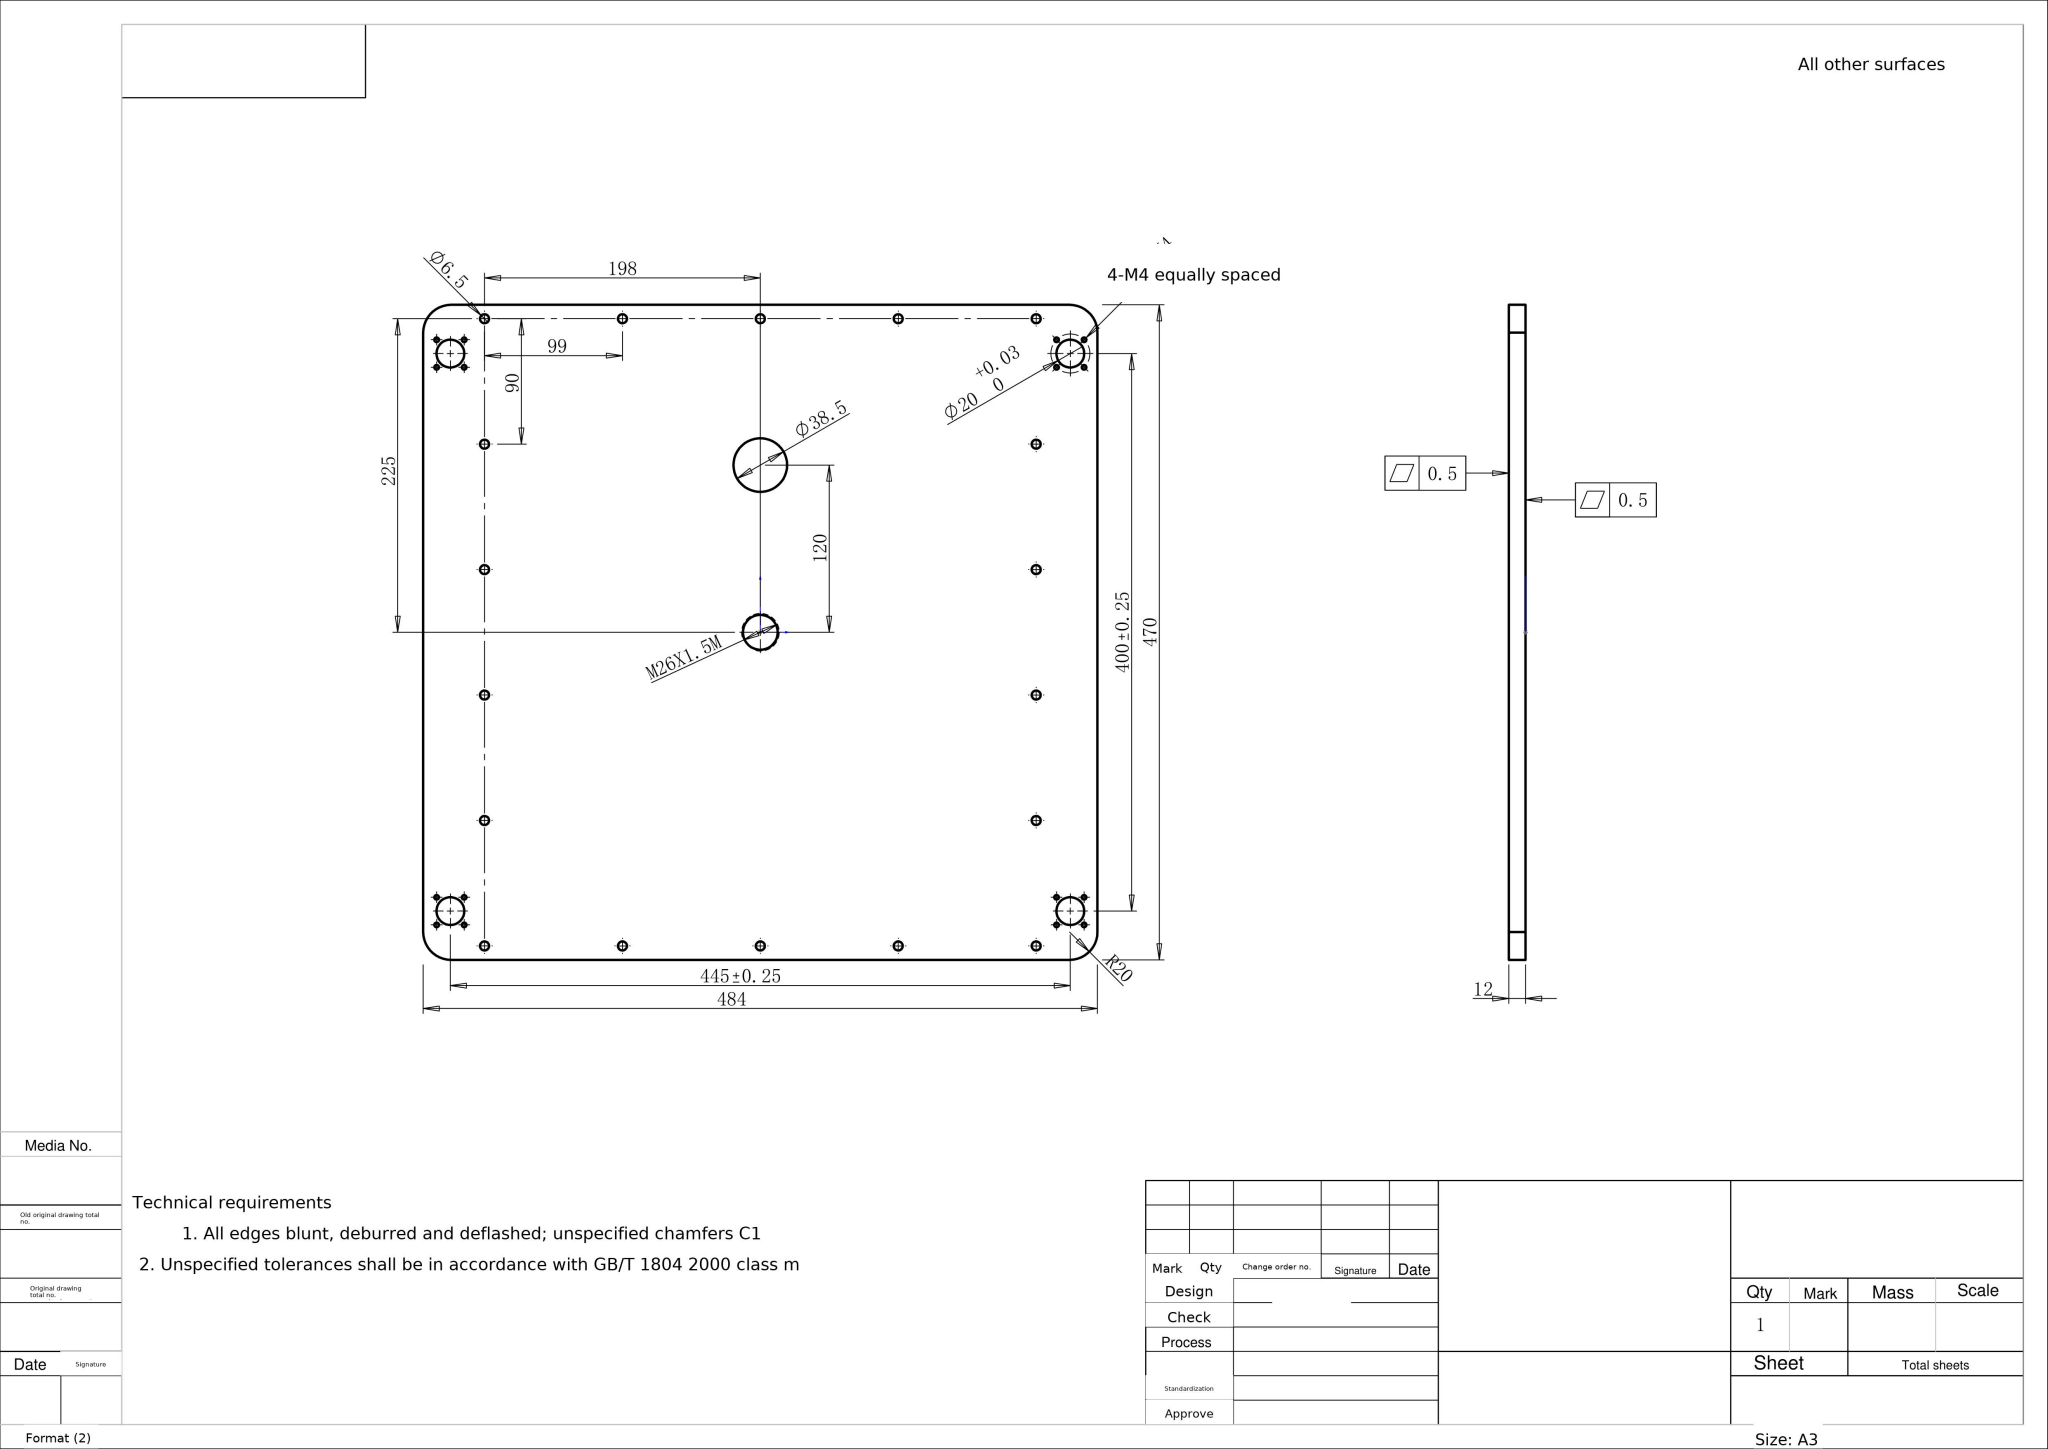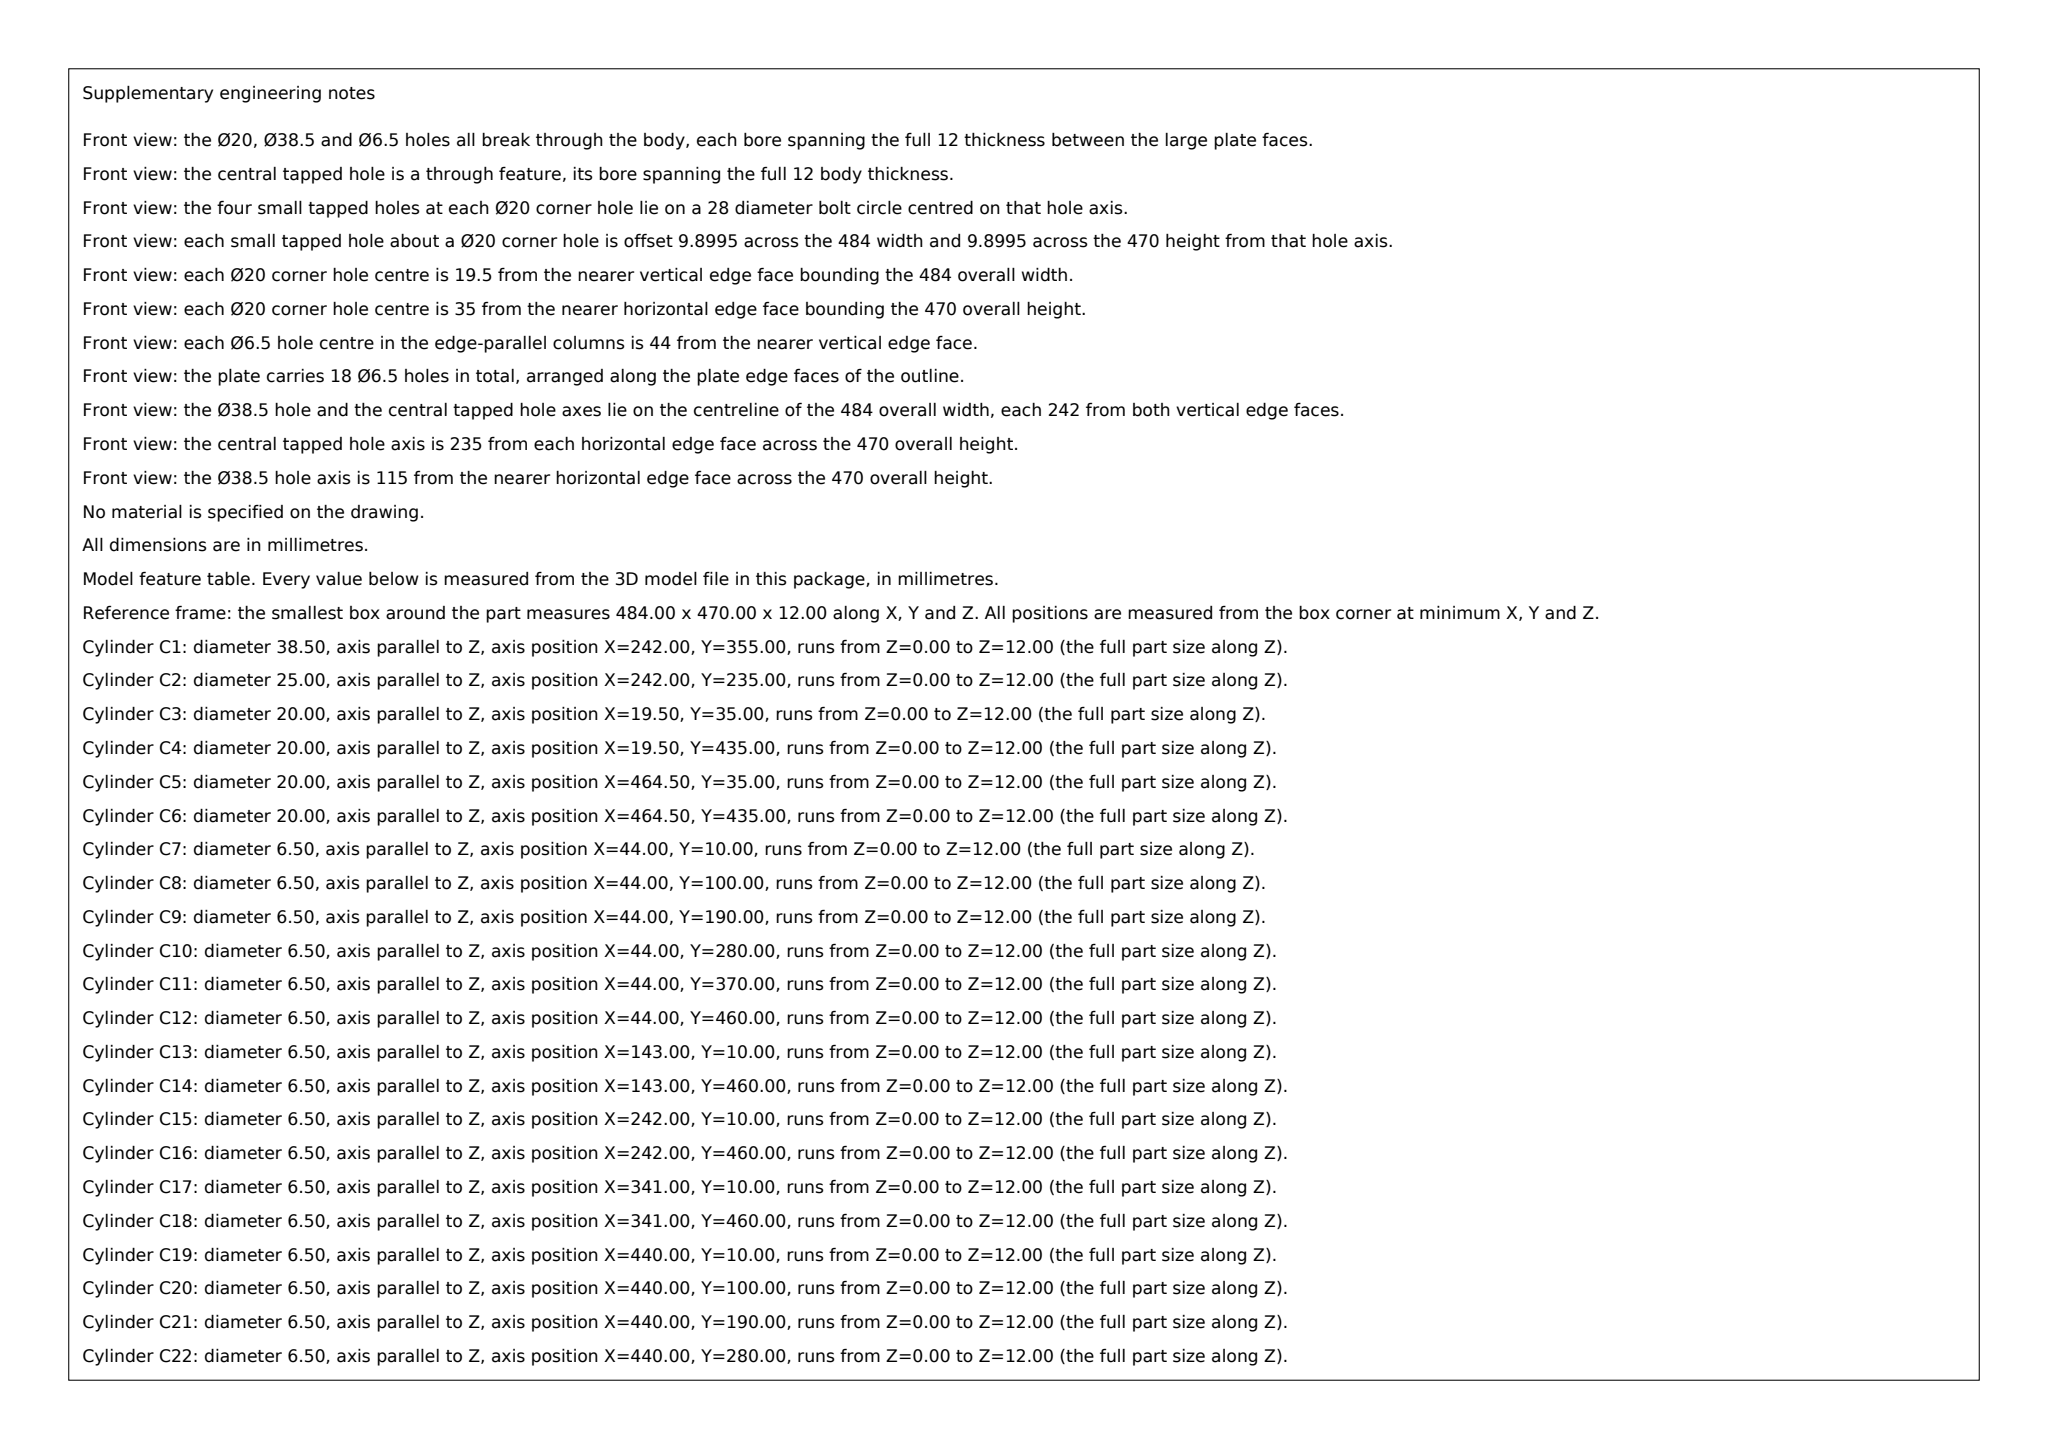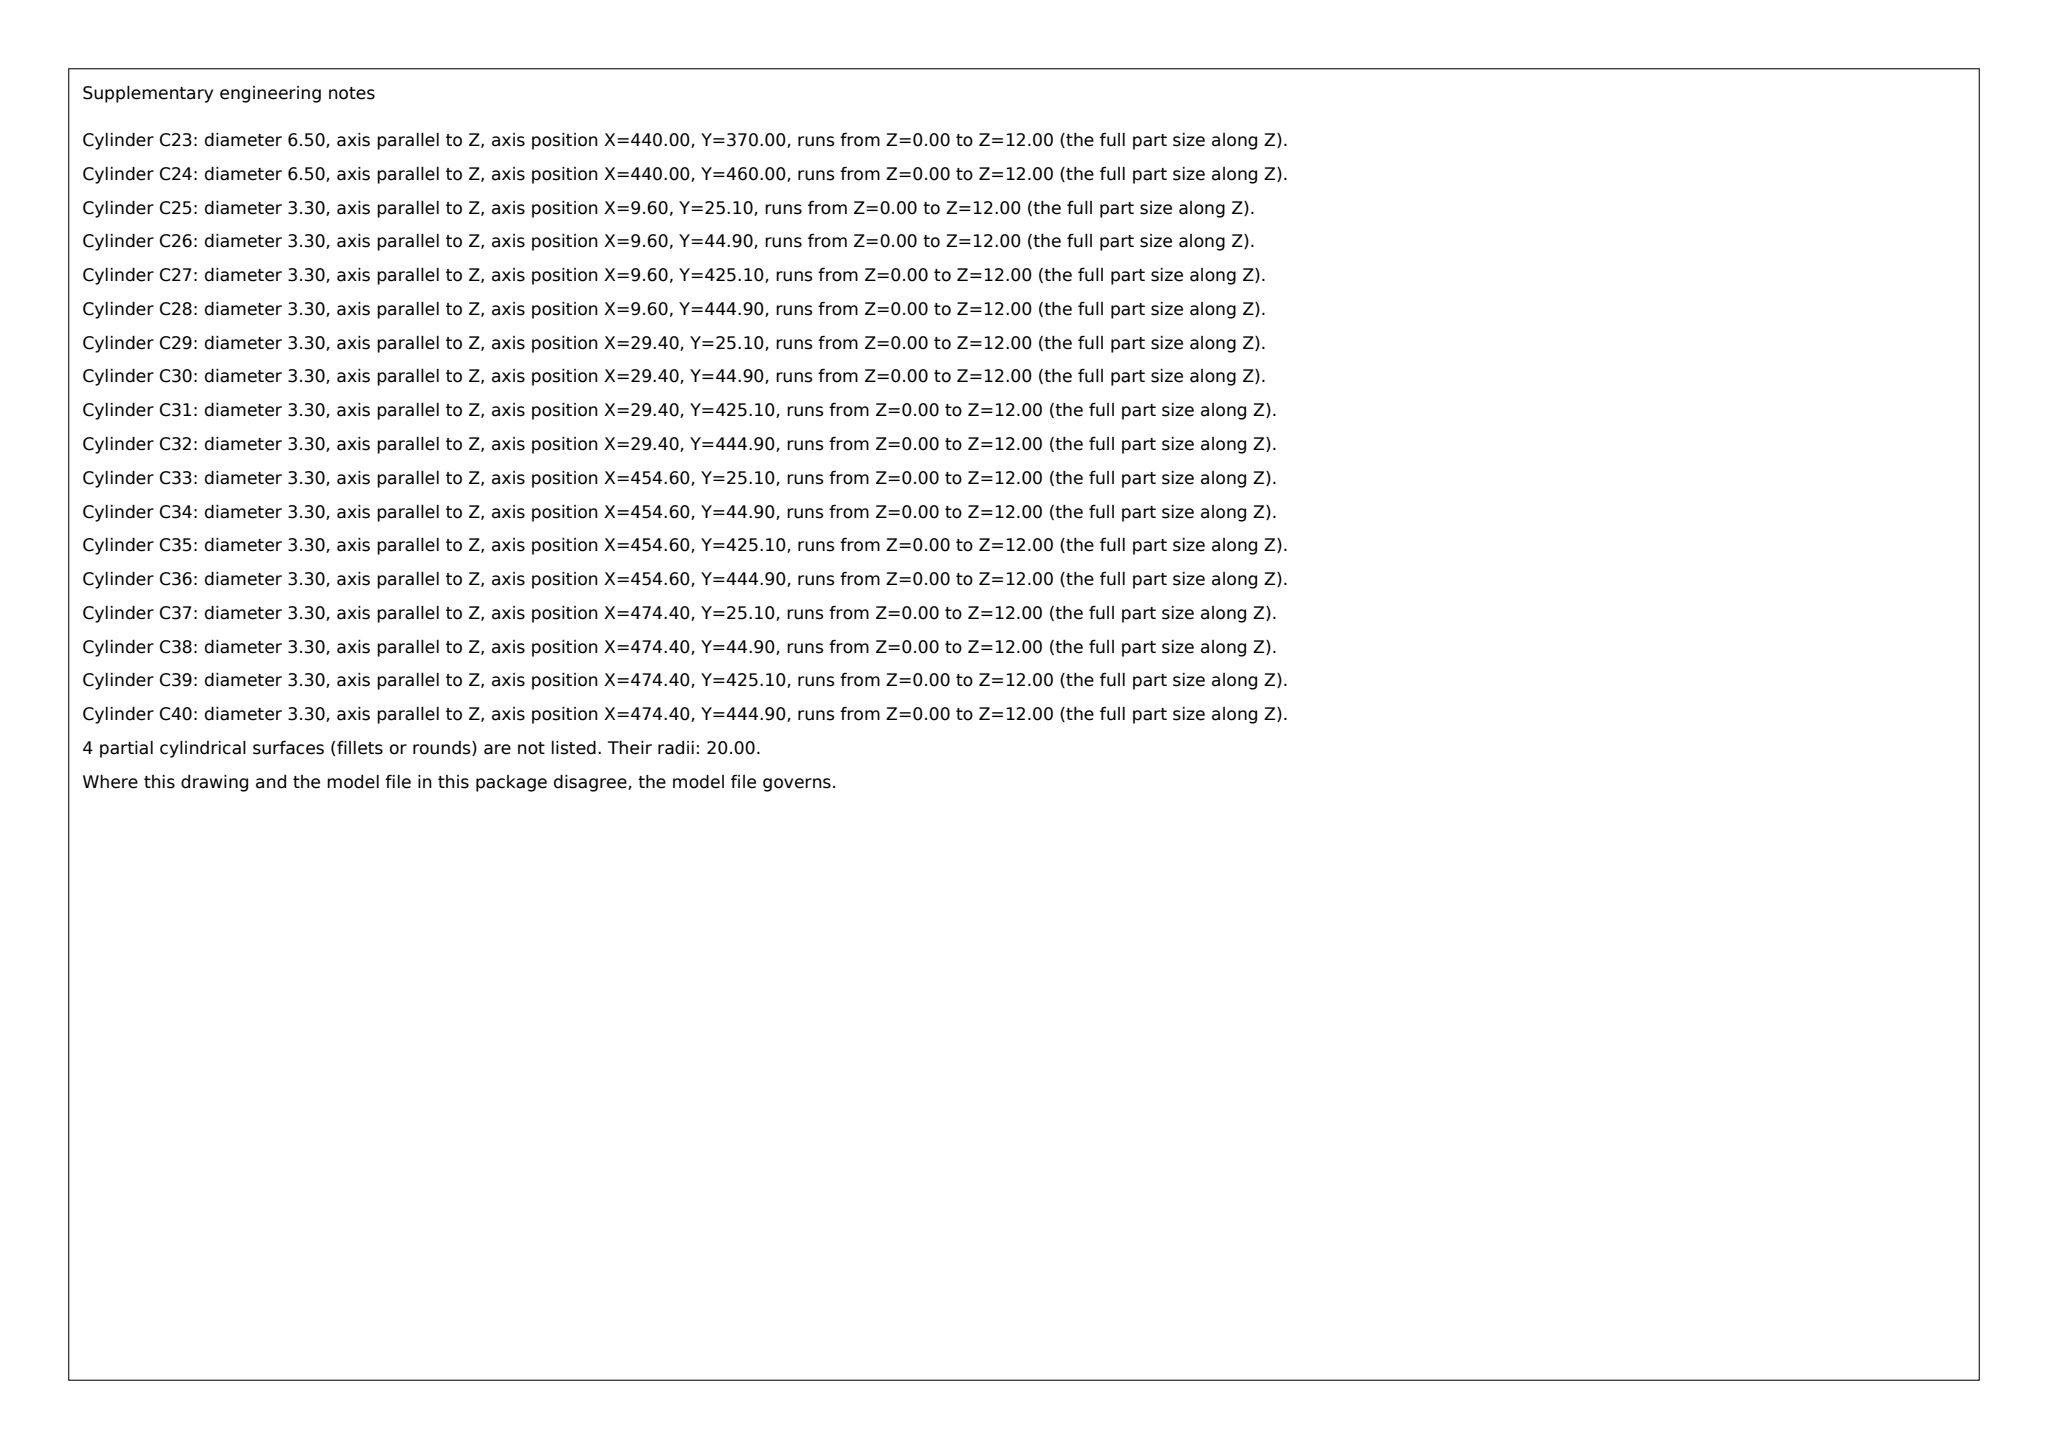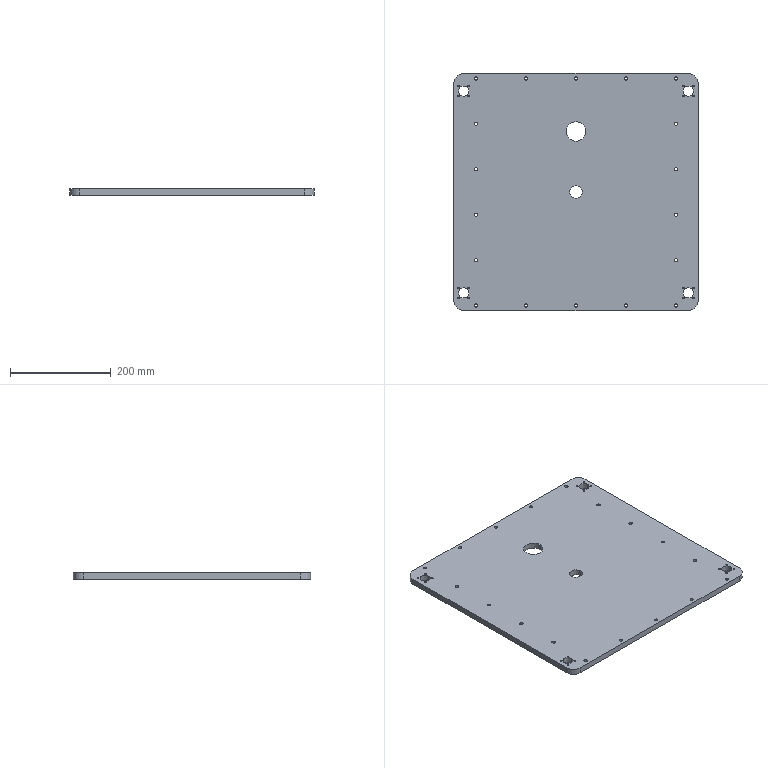Part | SolidWorks | mm | 1 solid | 90 faces | box 484 x 470 x 12 mm | volume 2681890 mm3 | cylinder 84 | plane 6 | commonest cylinder face diameters 6.5 x36 3.3 x32 20 x8 40 x4 38.5 x2 25 x2
Drawing notes:
Ø6.5 PATTERN: 44 FROM EA SIDE EDGE, 10 FROM EA TOP/BTM EDGE | from the solid: Ø6.5 cyls at x=44 & 440 (484-44), y=10 & 460 (470-10)
M26X1.5 ON PLATE CL: 242 FROM SIDE EDGE, 235 FROM BTM EDGE | from the solid: Ø25 (M26x1.5) cyl at [242.0,235.0]; bbox 484x470
4-M4 EQ SP ON Ø28 B.C., AT 45° TO AXES (9.9 X & 9.9 Y) | from the solid: Ø3.3 holes at ±9.9 X/Y from each Ø20 center, e.g. 19.5,35 -> 9.6/29.4, 25.1/44.9
ALL HOLES THRU 12 PLATE, INCL 4-M4 & M26X1.5 | from the solid: all cylinders length=12.0 = plate thickness (z planes 0 & 12)